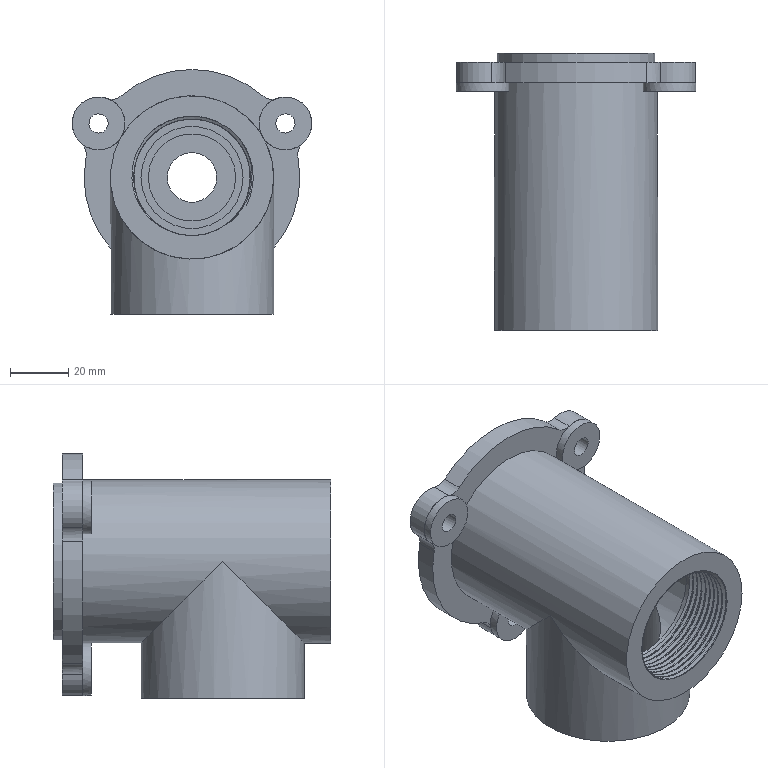Component | NX | 1 | 1 solid | 60 faces | volume 157253 mm3 | cylinder 33 | plane 24 | spline 2 | cone 1 | commonest cylinder face diameters 10 x6 4 x4 74 x3 18 x3 18.1 x3 6.6 x3 56 x2 30 x2